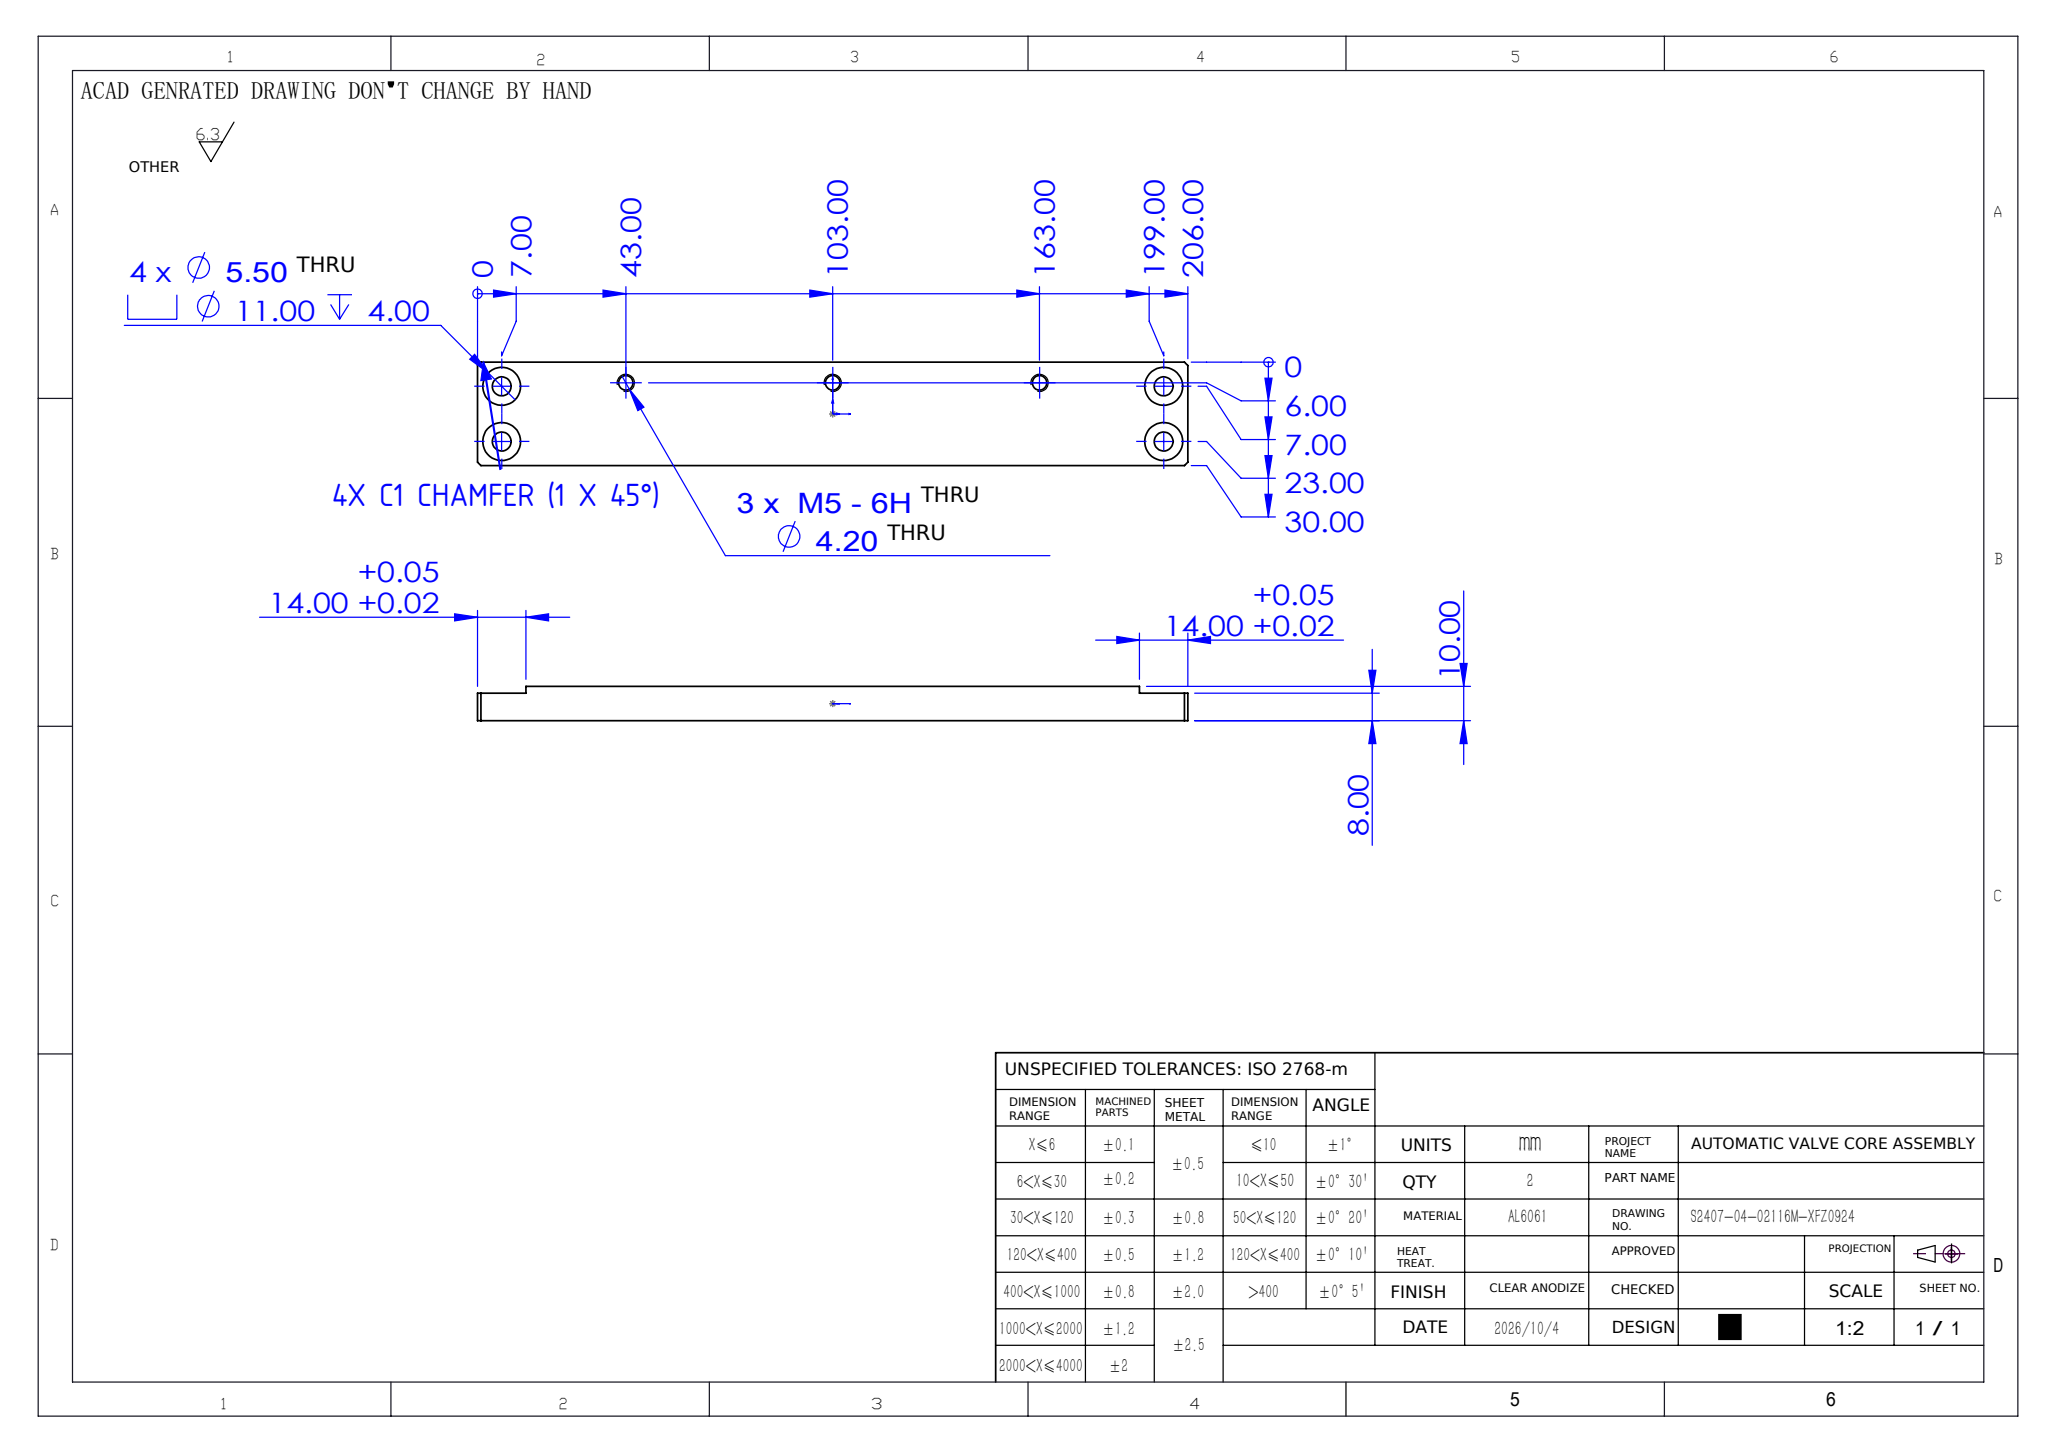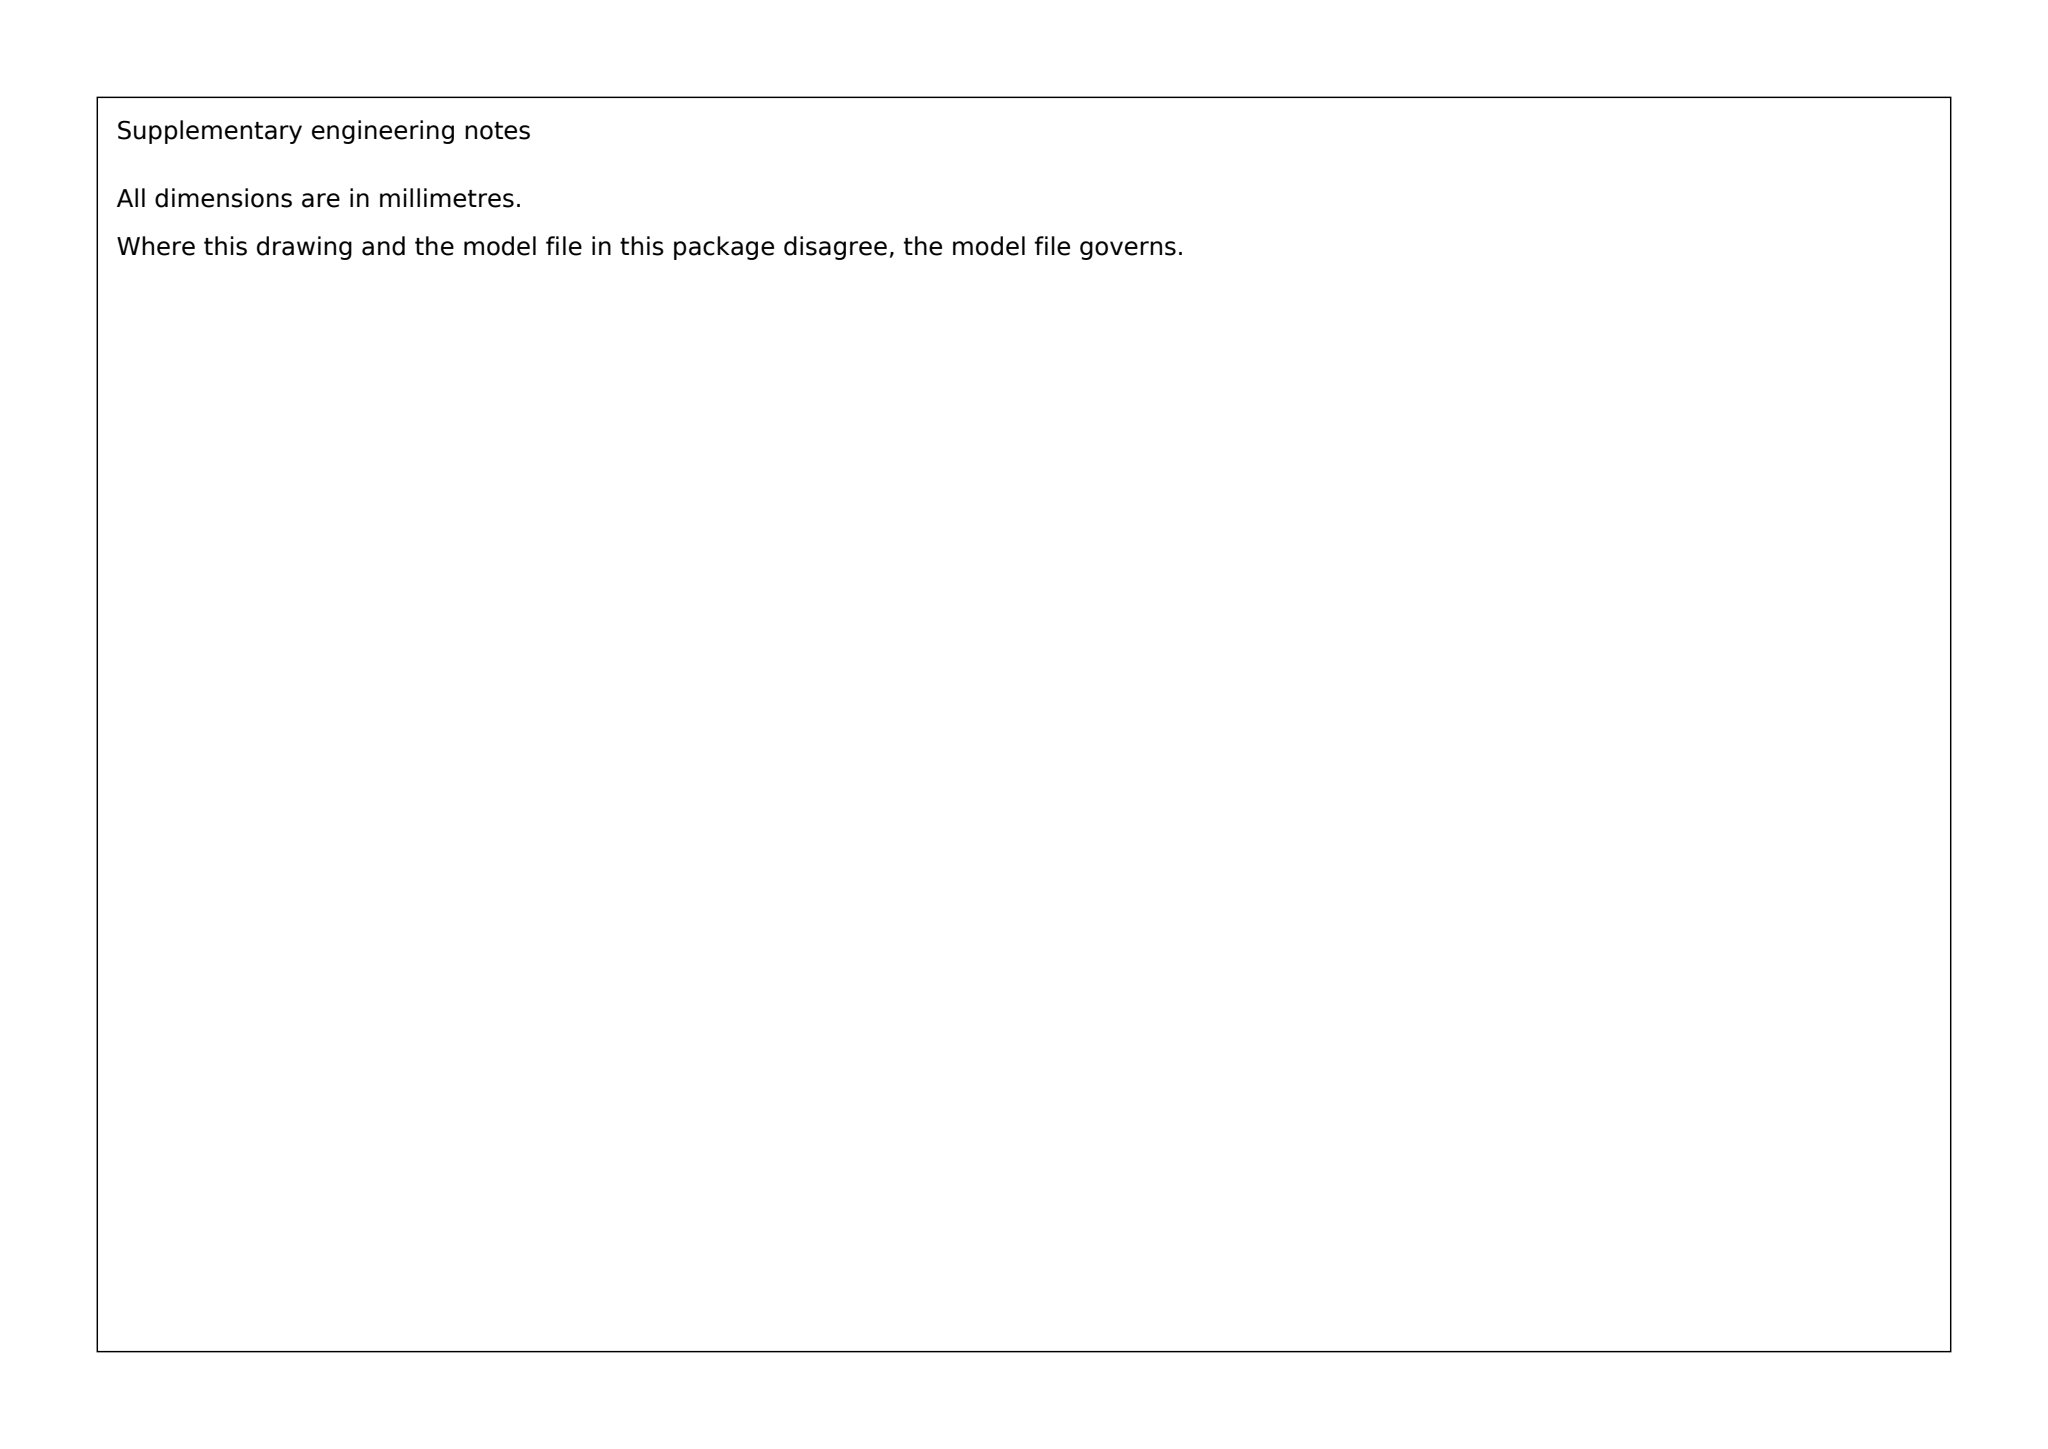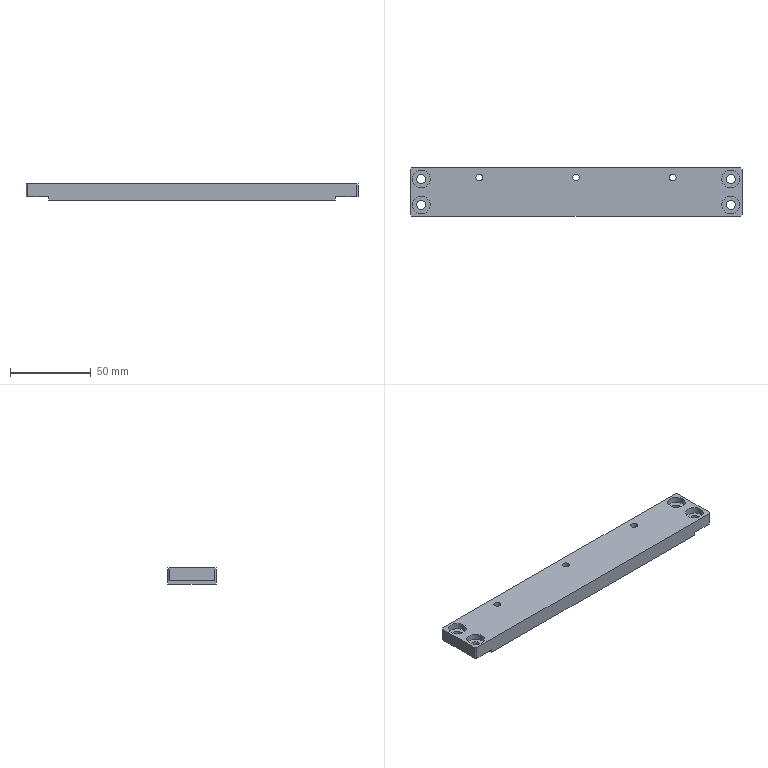Part | SolidWorks | mm | material AL6061 | 1 solid | 40 faces | box 206 x 30 x 10 mm | volume 57788 mm3 | cylinder 22 | plane 18 | commonest cylinder face diameters 11 x8 5.5 x8 4.2 x6
Drawing notes:
4X CORNER CHAMFER C1 (1 X 45°), FROM 2 ABOVE BOTTOM TO TOP | from the solid: 4 inclined planes 45°/45°, bbox_from z=2, size [1,1,8] at x=0/205, y=0/29
build123d program:
from build123d import *

# Parameters (mm, degrees)
SKETCH1_W                                          = 206
SKETCH1_H                                          = 30
BOSS_EXTRUDE1_DEPTH                                = 5
M5_TAPPED_HOLE1_D                                  = 4.2
SKETCH4_W                                          = 14
SKETCH4_H                                          = 30
CUT_EXTRUDE1_DEPTH                                 = 2
HOLE_SIZE_ACCORDING_TO_TYPE_1_OF_HEXAG_D           = 5.5
HOLE_SIZE_ACCORDING_TO_TYPE_1_OF_HEXAG_CBORE_D     = 11
HOLE_SIZE_ACCORDING_TO_TYPE_1_OF_HEXAG_CBORE_DEPTH = 4
CHAMFER1_SIZE                                      = 1


with BuildPart() as part:
    # Sketch1 → Boss-Extrude1 (new, symmetric)
    with BuildSketch(Plane.XY):
        Rectangle(SKETCH1_W, SKETCH1_H)
    extrude(amount=BOSS_EXTRUDE1_DEPTH, both=True)

    # M5 Tapped Hole1 (through all)
    with Locations(Plane.XY.offset(5)):
        with Locations((0, 9), (-60, 9), (60, 9)):
            Hole(M5_TAPPED_HOLE1_D / 2)

    # Sketch4 → Cut-Extrude1 (cut)
    with BuildSketch(Plane(origin=(0, 0, -5), x_dir=(-1, 0, 0), z_dir=(0, 0, -1))):
        with Locations((-96, 0)):
            Rectangle(SKETCH4_W, SKETCH4_H)
        with Locations((96, 0)):
            Rectangle(SKETCH4_W, SKETCH4_H)
    extrude(amount=-CUT_EXTRUDE1_DEPTH, mode=Mode.SUBTRACT)

    # Hole Size _According to_ Type 1 of Hexag (through all)
    with Locations(Plane.XY.offset(5)):
        with Locations((96, 8), (-96, 8), (-96, -8), (96, -8)):
            CounterBoreHole(HOLE_SIZE_ACCORDING_TO_TYPE_1_OF_HEXAG_D / 2, HOLE_SIZE_ACCORDING_TO_TYPE_1_OF_HEXAG_CBORE_D / 2, HOLE_SIZE_ACCORDING_TO_TYPE_1_OF_HEXAG_CBORE_DEPTH)

    # Chamfer1
    chamfer1_edges = [part.edges().sort_by_distance(p)[0] for p in [
        (103, -15, 1),
        (-103, -15, 1),
        (-103, 15, 1),
        (103, 15, 1),
    ]]
    chamfer(chamfer1_edges, length=CHAMFER1_SIZE)


solid = part.part